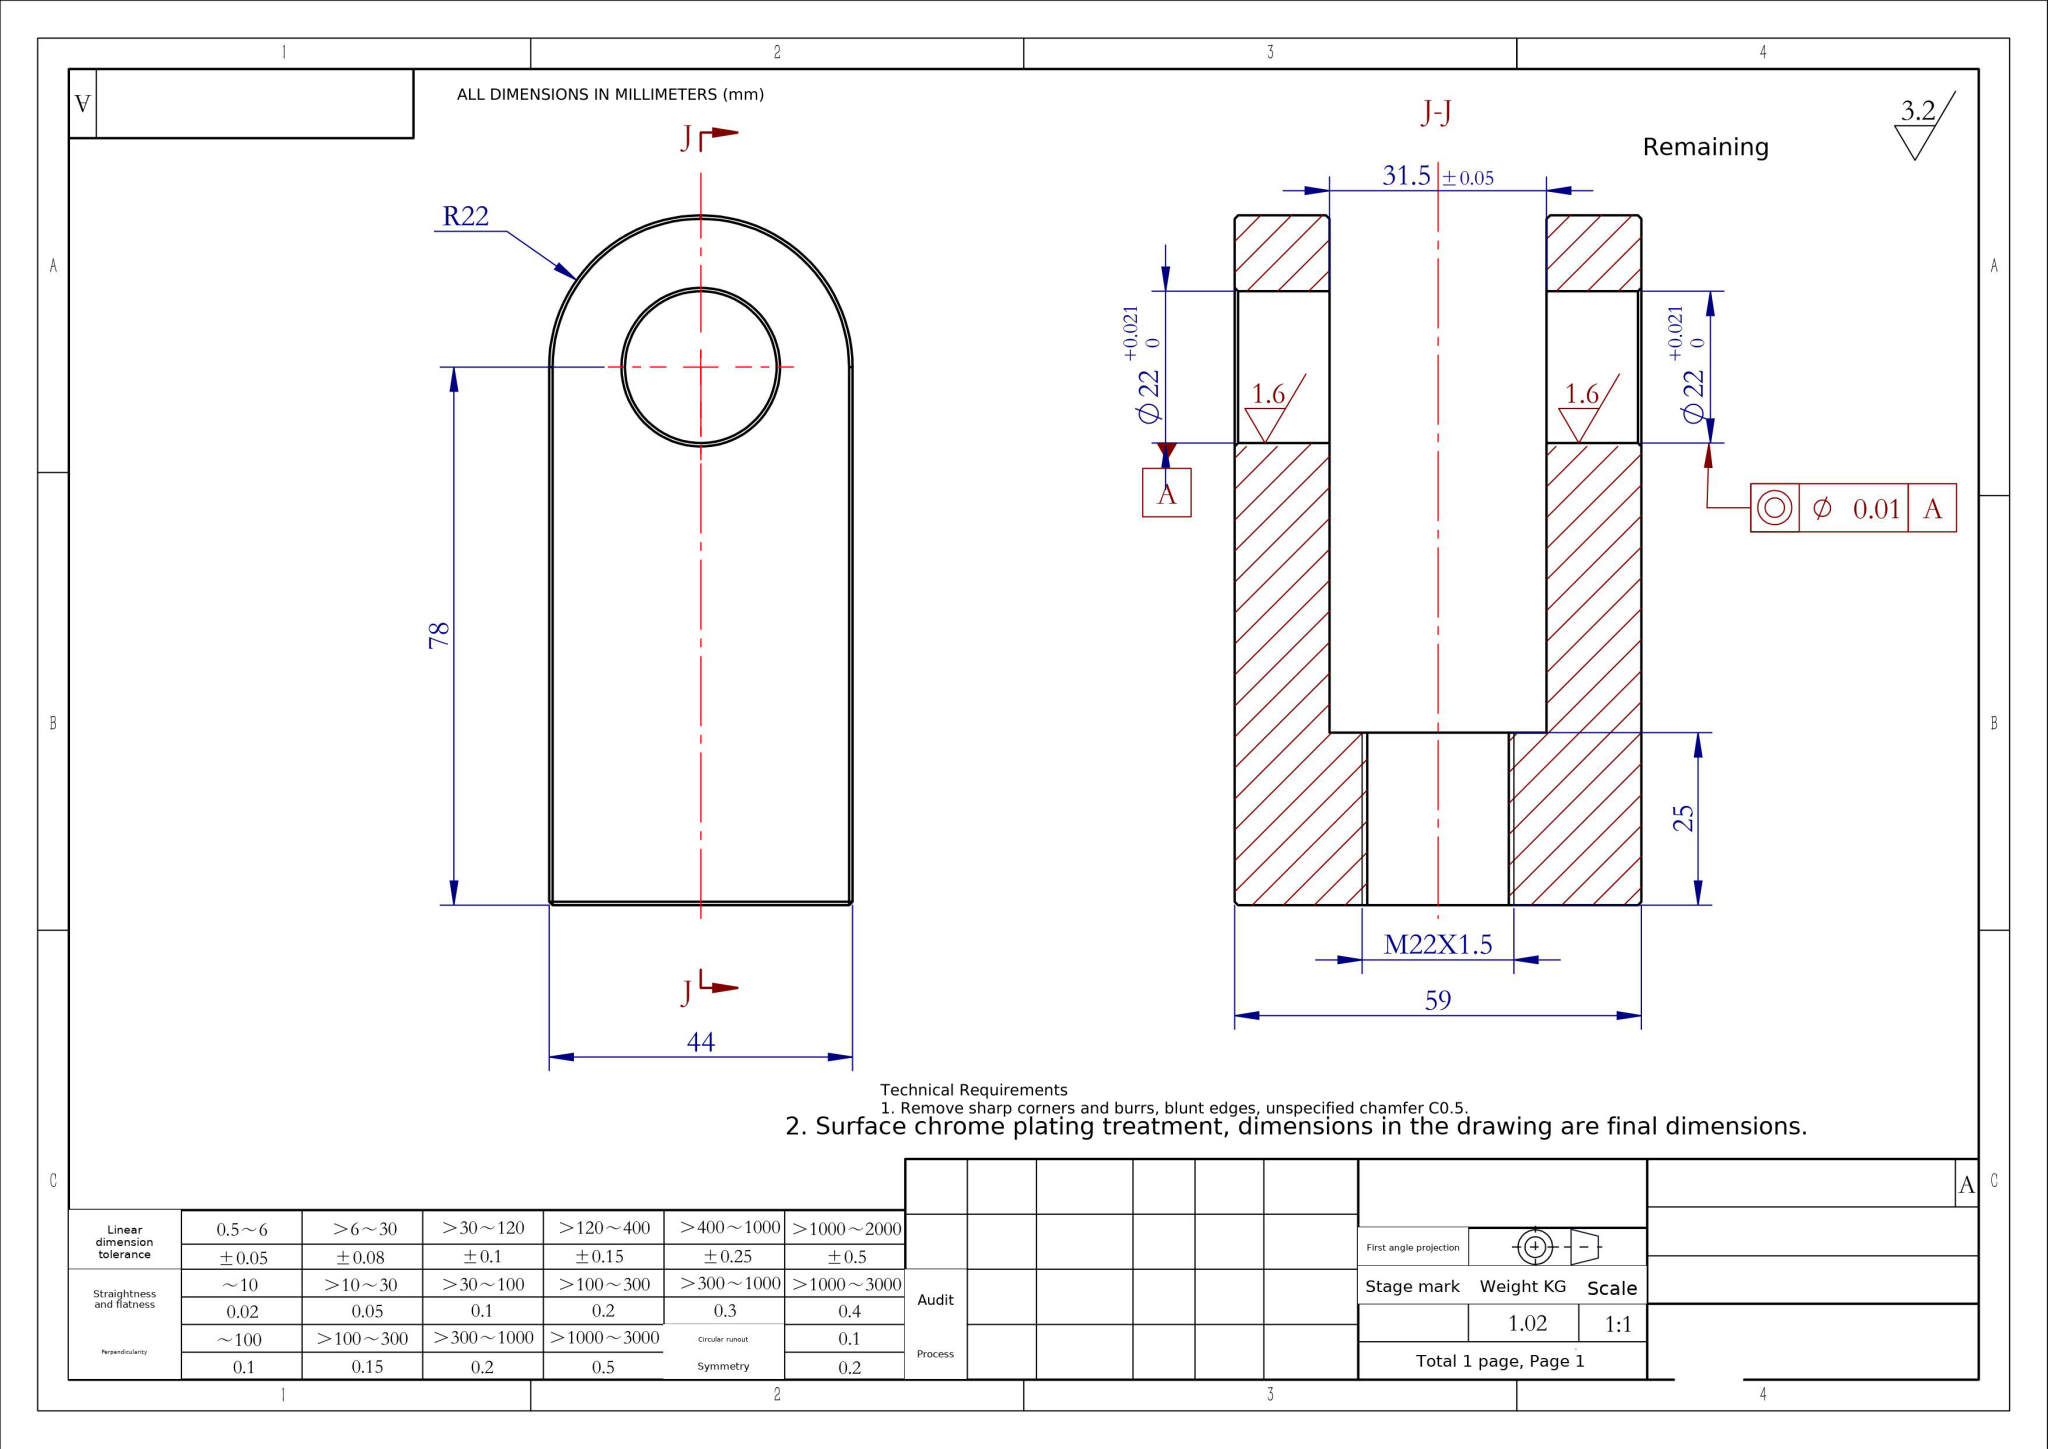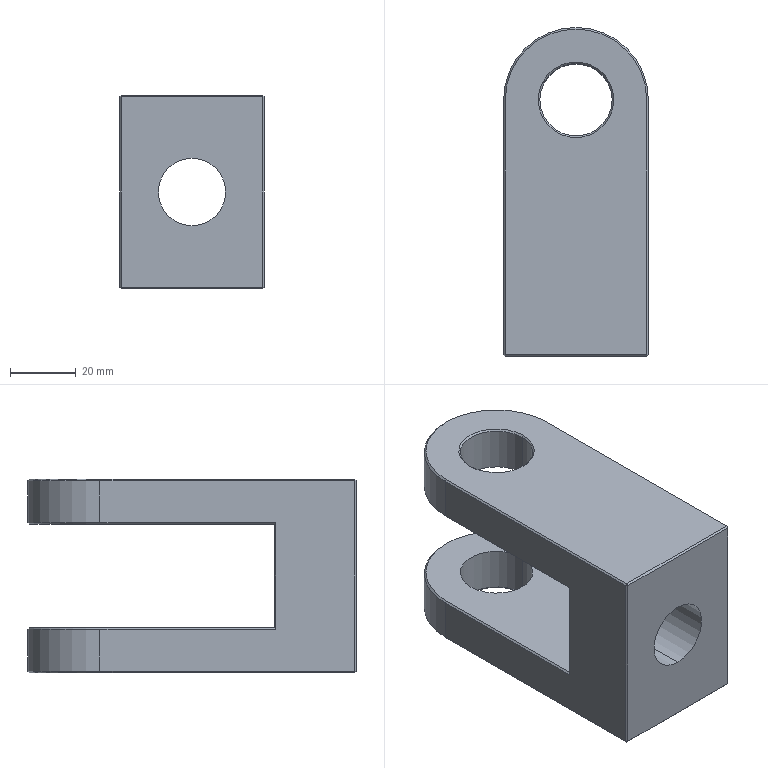Part | NX | mm | 1 solid | 48 faces | box 44 x 100 x 59 mm | volume 131081 mm3 | plane 26 | cone 12 | cylinder 10 | commonest cylinder face diameters 22 x4 44 x4 20.5 x2